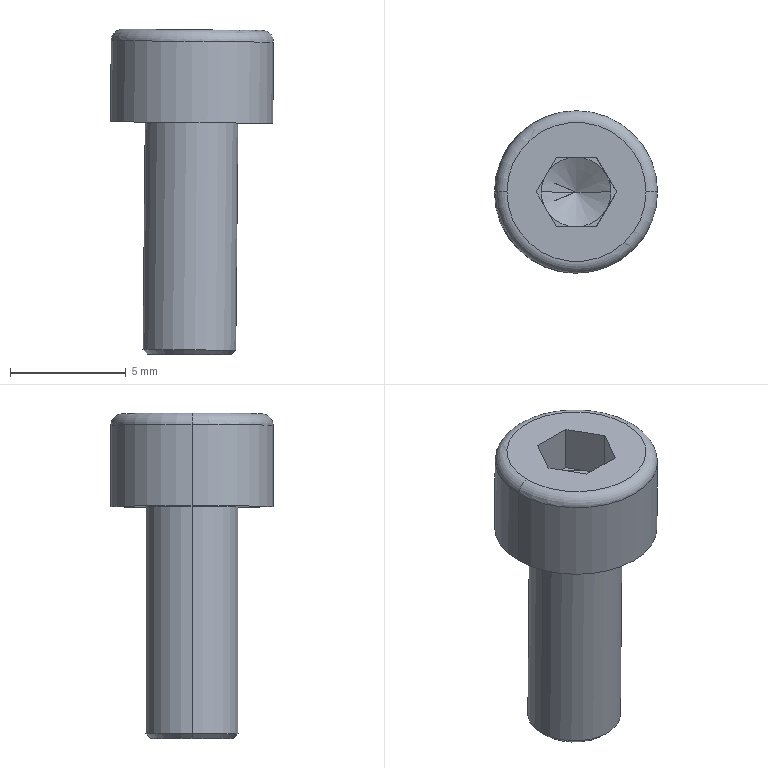Component | SolidWorks | hexagon socket head cap screws gb-14 | 1 solid | 25 faces | box 7.03 x 7 x 14.05 mm | volume 261 mm3 | plane 15 | cone 4 | cylinder 4 | torus 2 | commonest cylinder face diameters 4 x2 7 x2
STEP:
#1=CARTESIAN_POINT('',(-0.8105,1.397,-0.0293));
#2=VERTEX_POINT('',#1);
#3=CARTESIAN_POINT('',(-0.6688,1.397,-0.03069));
#4=VERTEX_POINT('',#3);
#5=CARTESIAN_POINT('',(-0.7397,1.397,-0.03));
#6=DIRECTION('',(-0.009793,0.,-1.));
#7=DIRECTION('',(-1.,0.,0.009793));
#8=AXIS2_PLACEMENT_3D('',#5,#6,#7);
#9=CIRCLE('',#8,0.07087);
#10=EDGE_CURVE('',#2,#4,#9,.T.);
#11=ORIENTED_EDGE('',*,*,#10,.F.);
#12=CARTESIAN_POINT('',(-0.8183,1.397,-0.02135));
#13=VERTEX_POINT('',#12);
#14=CARTESIAN_POINT('',(-0.8105,1.397,-0.0293));
#15=DIRECTION('',(-0.7001,-0.,0.714));
#16=VECTOR('',#15,39.37);
#17=LINE('',#14,#16);
#18=EDGE_CURVE('',#2,#13,#17,.T.);
#19=ORIENTED_EDGE('',*,*,#18,.T.);
#20=CARTESIAN_POINT('',(-0.6609,1.397,-0.02289));
#21=VERTEX_POINT('',#20);
#22=CARTESIAN_POINT('',(-0.7396,1.397,-0.02212));
#23=DIRECTION('',(0.009793,-0.,1.));
#24=DIRECTION('',(-1.,0.,0.009793));
#25=AXIS2_PLACEMENT_3D('',#22,#23,#24);
#26=CIRCLE('',#25,0.07874);
#27=EDGE_CURVE('',#21,#13,#26,.T.);
#28=ORIENTED_EDGE('',*,*,#27,.F.);
#29=CARTESIAN_POINT('',(-0.6688,1.397,-0.03069));
#30=DIRECTION('',(0.714,-0.,0.7001));
#31=VECTOR('',#30,39.37);
#32=LINE('',#29,#31);
#33=EDGE_CURVE('',#4,#21,#32,.T.);
#34=ORIENTED_EDGE('',*,*,#33,.F.);
#35=EDGE_LOOP('',(#11,#19,#28,#34));
#36=FACE_OUTER_BOUND('',#35,.T.);
#37=CARTESIAN_POINT('',(-0.7397,1.397,-0.03));
#38=DIRECTION('',(0.009793,-0.,1.));
#39=DIRECTION('',(1.,0.,-0.009793));
#40=AXIS2_PLACEMENT_3D('',#37,#38,#39);
#41=CONICAL_SURFACE('',#40,0.07087,0.7854);
#42=ADVANCED_FACE('',(#36),#41,.T.);
#43=CARTESIAN_POINT('',(-0.6162,1.397,0.52));
#44=VERTEX_POINT('',#43);
#45=CARTESIAN_POINT('',(-0.8524,1.397,0.5223));
#46=VERTEX_POINT('',#45);
#47=CARTESIAN_POINT('',(-0.7343,1.397,0.5212));
#48=DIRECTION('',(0.009793,-0.,1.));
#49=DIRECTION('',(-1.,0.,0.009793));
#50=AXIS2_PLACEMENT_3D('',#47,#48,#49);
#51=CIRCLE('',#50,0.1181);
#52=EDGE_CURVE('',#44,#46,#51,.T.);
#53=ORIENTED_EDGE('',*,*,#52,.F.);
#54=CARTESIAN_POINT('',(-0.5967,1.397,0.5001));
#55=VERTEX_POINT('',#54);
#56=CARTESIAN_POINT('',(-0.6164,1.397,0.5003));
#57=DIRECTION('',(-0.,1.,0.));
#58=DIRECTION('',(0.,0.,1.));
#59=AXIS2_PLACEMENT_3D('',#56,#57,#58);
#60=CIRCLE('',#59,0.01969);
#61=EDGE_CURVE('',#44,#55,#60,.T.);
#62=ORIENTED_EDGE('',*,*,#61,.T.);
#63=CARTESIAN_POINT('',(-0.8723,1.397,0.5028));
#64=VERTEX_POINT('',#63);
#65=CARTESIAN_POINT('',(-0.7345,1.397,0.5015));
#66=DIRECTION('',(-0.009793,0.,-1.));
#67=DIRECTION('',(-1.,0.,0.009793));
#68=AXIS2_PLACEMENT_3D('',#65,#66,#67);
#69=CIRCLE('',#68,0.1378);
#70=EDGE_CURVE('',#64,#55,#69,.T.);
#71=ORIENTED_EDGE('',*,*,#70,.F.);
#72=CARTESIAN_POINT('',(-0.8526,1.397,0.5026));
#73=DIRECTION('',(0.,-1.,-0.));
#74=DIRECTION('',(0.,0.,-1.));
#75=AXIS2_PLACEMENT_3D('',#72,#73,#74);
#76=CIRCLE('',#75,0.01969);
#77=EDGE_CURVE('',#46,#64,#76,.T.);
#78=ORIENTED_EDGE('',*,*,#77,.F.);
#79=EDGE_LOOP('',(#53,#62,#71,#78));
#80=FACE_OUTER_BOUND('',#79,.T.);
#81=CARTESIAN_POINT('',(-0.7345,1.397,0.5015));
#82=DIRECTION('',(-0.009793,0.,-1.));
#83=DIRECTION('',(-1.,0.,0.009793));
#84=AXIS2_PLACEMENT_3D('',#81,#82,#83);
#85=TOROIDAL_SURFACE('',#84,0.1181,0.01969);
#86=ADVANCED_FACE('',(#80),#85,.T.);
#87=CARTESIAN_POINT('',(-0.7354,1.397,0.4083));
#88=VERTEX_POINT('',#87);
#89=CARTESIAN_POINT('',(-0.676,1.397,0.4418));
#90=VERTEX_POINT('',#89);
#91=CARTESIAN_POINT('',(-0.676,1.397,0.4418));
#92=DIRECTION('',(0.8709,-0.,0.4915));
#93=VECTOR('',#92,39.37);
#94=LINE('',#91,#93);
#95=EDGE_CURVE('',#88,#90,#94,.T.);
#96=ORIENTED_EDGE('',*,*,#95,.F.);
#97=CARTESIAN_POINT('',(-0.7941,1.397,0.443));
#98=VERTEX_POINT('',#97);
#99=CARTESIAN_POINT('',(-0.7941,1.397,0.443));
#100=DIRECTION('',(-0.8611,-0.,0.5085));
#101=VECTOR('',#100,39.37);
#102=LINE('',#99,#101);
#103=EDGE_CURVE('',#88,#98,#102,.T.);
#104=ORIENTED_EDGE('',*,*,#103,.T.);
#105=CARTESIAN_POINT('',(-0.7862,1.368,0.4429));
#106=VERTEX_POINT('',#105);
#107=CARTESIAN_POINT('',(-0.7351,1.397,0.4424));
#108=DIRECTION('',(-0.009793,0.,-1.));
#109=DIRECTION('',(1.,0.,-0.009793));
#110=AXIS2_PLACEMENT_3D('',#107,#108,#109);
#111=CIRCLE('',#110,0.05906);
#112=EDGE_CURVE('',#106,#98,#111,.T.);
#113=ORIENTED_EDGE('',*,*,#112,.F.);
#114=CARTESIAN_POINT('',(-0.7351,1.338,0.4424));
#115=VERTEX_POINT('',#114);
#116=CARTESIAN_POINT('',(-0.7351,1.397,0.4424));
#117=DIRECTION('',(-0.009793,0.,-1.));
#118=DIRECTION('',(1.,0.,-0.009793));
#119=AXIS2_PLACEMENT_3D('',#116,#117,#118);
#120=CIRCLE('',#119,0.05906);
#121=EDGE_CURVE('',#115,#106,#120,.T.);
#122=ORIENTED_EDGE('',*,*,#121,.F.);
#123=CARTESIAN_POINT('',(-0.6839,1.368,0.4419));
#124=VERTEX_POINT('',#123);
#125=CARTESIAN_POINT('',(-0.7351,1.397,0.4424));
#126=DIRECTION('',(-0.009793,0.,-1.));
#127=DIRECTION('',(1.,0.,-0.009793));
#128=AXIS2_PLACEMENT_3D('',#125,#126,#127);
#129=CIRCLE('',#128,0.05906);
#130=EDGE_CURVE('',#124,#115,#129,.T.);
#131=ORIENTED_EDGE('',*,*,#130,.F.);
#132=CARTESIAN_POINT('',(-0.7351,1.397,0.4424));
#133=DIRECTION('',(-0.009793,0.,-1.));
#134=DIRECTION('',(1.,0.,-0.009793));
#135=AXIS2_PLACEMENT_3D('',#132,#133,#134);
#136=CIRCLE('',#135,0.05906);
#137=EDGE_CURVE('',#90,#124,#136,.T.);
#138=ORIENTED_EDGE('',*,*,#137,.F.);
#139=EDGE_LOOP('',(#96,#104,#113,#122,#131,#138));
#140=FACE_OUTER_BOUND('',#139,.T.);
#141=CARTESIAN_POINT('',(-0.7351,1.397,0.4424));
#142=DIRECTION('',(0.009793,-0.,1.));
#143=DIRECTION('',(1.,0.,-0.009793));
#144=AXIS2_PLACEMENT_3D('',#141,#142,#143);
#145=CONICAL_SURFACE('',#144,0.05906,1.047);
#146=ADVANCED_FACE('',(#140),#145,.F.);
#147=ORIENTED_EDGE('',*,*,#27,.T.);
#148=CARTESIAN_POINT('',(-0.8146,1.397,0.3645));
#149=VERTEX_POINT('',#148);
#150=CARTESIAN_POINT('',(-0.8184,1.397,-0.02923));
#151=DIRECTION('',(0.009793,-0.,1.));
#152=VECTOR('',#151,39.37);
#153=LINE('',#150,#152);
#154=EDGE_CURVE('',#13,#149,#153,.T.);
#155=ORIENTED_EDGE('',*,*,#154,.T.);
#156=CARTESIAN_POINT('',(-0.6571,1.397,0.3629));
#157=VERTEX_POINT('',#156);
#158=CARTESIAN_POINT('',(-0.7358,1.397,0.3637));
#159=DIRECTION('',(-0.009793,0.,-1.));
#160=DIRECTION('',(-1.,0.,0.009793));
#161=AXIS2_PLACEMENT_3D('',#158,#159,#160);
#162=CIRCLE('',#161,0.07874);
#163=EDGE_CURVE('',#149,#157,#162,.T.);
#164=ORIENTED_EDGE('',*,*,#163,.T.);
#165=CARTESIAN_POINT('',(-0.661,1.397,-0.03077));
#166=DIRECTION('',(0.009793,-0.,1.));
#167=VECTOR('',#166,39.37);
#168=LINE('',#165,#167);
#169=EDGE_CURVE('',#21,#157,#168,.T.);
#170=ORIENTED_EDGE('',*,*,#169,.F.);
#171=EDGE_LOOP('',(#147,#155,#164,#170));
#172=FACE_OUTER_BOUND('',#171,.T.);
#173=CARTESIAN_POINT('',(-0.7397,1.397,-0.03));
#174=DIRECTION('',(0.009793,-0.,1.));
#175=DIRECTION('',(1.,0.,-0.009793));
#176=AXIS2_PLACEMENT_3D('',#173,#174,#175);
#177=CYLINDRICAL_SURFACE('',#176,0.07874);
#178=ADVANCED_FACE('',(#172),#177,.T.);
#179=CARTESIAN_POINT('',(-0.8736,1.397,0.365));
#180=VERTEX_POINT('',#179);
#181=CARTESIAN_POINT('',(-0.598,1.397,0.3623));
#182=VERTEX_POINT('',#181);
#183=CARTESIAN_POINT('',(-0.7358,1.397,0.3637));
#184=DIRECTION('',(-0.009793,0.,-1.));
#185=DIRECTION('',(-1.,0.,0.009793));
#186=AXIS2_PLACEMENT_3D('',#183,#184,#185);
#187=CIRCLE('',#186,0.1378);
#188=EDGE_CURVE('',#180,#182,#187,.T.);
#189=ORIENTED_EDGE('',*,*,#188,.F.);
#190=CARTESIAN_POINT('',(-0.8736,1.397,0.365));
#191=DIRECTION('',(0.009793,-0.,1.));
#192=VECTOR('',#191,39.37);
#193=LINE('',#190,#192);
#194=EDGE_CURVE('',#180,#64,#193,.T.);
#195=ORIENTED_EDGE('',*,*,#194,.T.);
#196=ORIENTED_EDGE('',*,*,#70,.T.);
#197=CARTESIAN_POINT('',(-0.598,1.397,0.3623));
#198=DIRECTION('',(0.009793,-0.,1.));
#199=VECTOR('',#198,39.37);
#200=LINE('',#197,#199);
#201=EDGE_CURVE('',#182,#55,#200,.T.);
#202=ORIENTED_EDGE('',*,*,#201,.F.);
#203=EDGE_LOOP('',(#189,#195,#196,#202));
#204=FACE_OUTER_BOUND('',#203,.T.);
#205=CARTESIAN_POINT('',(-0.7358,1.397,0.3637));
#206=DIRECTION('',(0.009793,-0.,1.));
#207=DIRECTION('',(1.,0.,-0.009793));
#208=AXIS2_PLACEMENT_3D('',#205,#206,#207);
#209=CYLINDRICAL_SURFACE('',#208,0.1378);
#210=ADVANCED_FACE('',(#204),#209,.T.);
#211=CARTESIAN_POINT('',(-0.701,1.338,0.4421));
#212=VERTEX_POINT('',#211);
#213=CARTESIAN_POINT('',(-0.6669,1.397,0.4418));
#214=DIRECTION('',(-0.5,-0.866,0.004897));
#215=VECTOR('',#214,39.37);
#216=LINE('',#213,#215);
#217=EDGE_CURVE('',#124,#212,#216,.T.);
#218=ORIENTED_EDGE('',*,*,#217,.F.);
#219=ORIENTED_EDGE('',*,*,#130,.T.);
#220=CARTESIAN_POINT('',(-0.701,1.338,0.4421));
#221=DIRECTION('',(-1.,-0.,0.009793));
#222=VECTOR('',#221,39.37);
#223=LINE('',#220,#222);
#224=EDGE_CURVE('',#212,#115,#223,.T.);
#225=ORIENTED_EDGE('',*,*,#224,.F.);
#226=EDGE_LOOP('',(#218,#219,#225));
#227=FACE_OUTER_BOUND('',#226,.T.);
#228=CARTESIAN_POINT('',(-0.7351,1.279,0.4424));
#229=DIRECTION('',(0.009793,-0.,1.));
#230=DIRECTION('',(1.,0.,-0.009793));
#231=AXIS2_PLACEMENT_3D('',#228,#229,#230);
#232=PLANE('',#231);
#233=ADVANCED_FACE('',(#227),#232,.T.);
#234=CARTESIAN_POINT('',(-0.7692,1.338,0.4428));
#235=VERTEX_POINT('',#234);
#236=CARTESIAN_POINT('',(-0.701,1.338,0.4421));
#237=DIRECTION('',(-1.,-0.,0.009793));
#238=VECTOR('',#237,39.37);
#239=LINE('',#236,#238);
#240=EDGE_CURVE('',#115,#235,#239,.T.);
#241=ORIENTED_EDGE('',*,*,#240,.F.);
#242=ORIENTED_EDGE('',*,*,#121,.T.);
#243=CARTESIAN_POINT('',(-0.7692,1.338,0.4428));
#244=DIRECTION('',(-0.5,0.866,0.004897));
#245=VECTOR('',#244,39.37);
#246=LINE('',#243,#245);
#247=EDGE_CURVE('',#235,#106,#246,.T.);
#248=ORIENTED_EDGE('',*,*,#247,.F.);
#249=EDGE_LOOP('',(#241,#242,#248));
#250=FACE_OUTER_BOUND('',#249,.T.);
#251=CARTESIAN_POINT('',(-0.7351,1.279,0.4424));
#252=DIRECTION('',(0.009793,-0.,1.));
#253=DIRECTION('',(1.,0.,-0.009793));
#254=AXIS2_PLACEMENT_3D('',#251,#252,#253);
#255=PLANE('',#254);
#256=ADVANCED_FACE('',(#250),#255,.T.);
#257=CARTESIAN_POINT('',(-0.8032,1.397,0.4431));
#258=VERTEX_POINT('',#257);
#259=CARTESIAN_POINT('',(-0.7692,1.338,0.4428));
#260=DIRECTION('',(-0.5,0.866,0.004897));
#261=VECTOR('',#260,39.37);
#262=LINE('',#259,#261);
#263=EDGE_CURVE('',#106,#258,#262,.T.);
#264=ORIENTED_EDGE('',*,*,#263,.F.);
#265=ORIENTED_EDGE('',*,*,#112,.T.);
#266=CARTESIAN_POINT('',(-0.7862,1.427,0.4429));
#267=VERTEX_POINT('',#266);
#268=CARTESIAN_POINT('',(-0.7351,1.397,0.4424));
#269=DIRECTION('',(-0.009793,0.,-1.));
#270=DIRECTION('',(1.,0.,-0.009793));
#271=AXIS2_PLACEMENT_3D('',#268,#269,#270);
#272=CIRCLE('',#271,0.05906);
#273=EDGE_CURVE('',#98,#267,#272,.T.);
#274=ORIENTED_EDGE('',*,*,#273,.T.);
#275=CARTESIAN_POINT('',(-0.8032,1.397,0.4431));
#276=DIRECTION('',(0.5,0.866,-0.004897));
#277=VECTOR('',#276,39.37);
#278=LINE('',#275,#277);
#279=EDGE_CURVE('',#258,#267,#278,.T.);
#280=ORIENTED_EDGE('',*,*,#279,.F.);
#281=EDGE_LOOP('',(#264,#265,#274,#280));
#282=FACE_OUTER_BOUND('',#281,.T.);
#283=CARTESIAN_POINT('',(-0.7351,1.279,0.4424));
#284=DIRECTION('',(0.009793,-0.,1.));
#285=DIRECTION('',(1.,0.,-0.009793));
#286=AXIS2_PLACEMENT_3D('',#283,#284,#285);
#287=PLANE('',#286);
#288=ADVANCED_FACE('',(#282),#287,.T.);
#289=CARTESIAN_POINT('',(-0.7692,1.456,0.4428));
#290=VERTEX_POINT('',#289);
#291=CARTESIAN_POINT('',(-0.8032,1.397,0.4431));
#292=DIRECTION('',(0.5,0.866,-0.004897));
#293=VECTOR('',#292,39.37);
#294=LINE('',#291,#293);
#295=EDGE_CURVE('',#267,#290,#294,.T.);
#296=ORIENTED_EDGE('',*,*,#295,.F.);
#297=CARTESIAN_POINT('',(-0.7351,1.456,0.4424));
#298=VERTEX_POINT('',#297);
#299=CARTESIAN_POINT('',(-0.7351,1.397,0.4424));
#300=DIRECTION('',(-0.009793,0.,-1.));
#301=DIRECTION('',(-1.,0.,0.009793));
#302=AXIS2_PLACEMENT_3D('',#299,#300,#301);
#303=CIRCLE('',#302,0.05906);
#304=EDGE_CURVE('',#267,#298,#303,.T.);
#305=ORIENTED_EDGE('',*,*,#304,.T.);
#306=CARTESIAN_POINT('',(-0.7692,1.456,0.4428));
#307=DIRECTION('',(1.,0.,-0.009793));
#308=VECTOR('',#307,39.37);
#309=LINE('',#306,#308);
#310=EDGE_CURVE('',#290,#298,#309,.T.);
#311=ORIENTED_EDGE('',*,*,#310,.F.);
#312=EDGE_LOOP('',(#296,#305,#311));
#313=FACE_OUTER_BOUND('',#312,.T.);
#314=CARTESIAN_POINT('',(-0.7351,1.279,0.4424));
#315=DIRECTION('',(0.009793,-0.,1.));
#316=DIRECTION('',(1.,0.,-0.009793));
#317=AXIS2_PLACEMENT_3D('',#314,#315,#316);
#318=PLANE('',#317);
#319=ADVANCED_FACE('',(#313),#318,.T.);
#320=CARTESIAN_POINT('',(-0.701,1.456,0.4421));
#321=VERTEX_POINT('',#320);
#322=CARTESIAN_POINT('',(-0.7692,1.456,0.4428));
#323=DIRECTION('',(1.,0.,-0.009793));
#324=VECTOR('',#323,39.37);
#325=LINE('',#322,#324);
#326=EDGE_CURVE('',#298,#321,#325,.T.);
#327=ORIENTED_EDGE('',*,*,#326,.F.);
#328=CARTESIAN_POINT('',(-0.6839,1.427,0.4419));
#329=VERTEX_POINT('',#328);
#330=CARTESIAN_POINT('',(-0.7351,1.397,0.4424));
#331=DIRECTION('',(-0.009793,0.,-1.));
#332=DIRECTION('',(1.,0.,-0.009793));
#333=AXIS2_PLACEMENT_3D('',#330,#331,#332);
#334=CIRCLE('',#333,0.05906);
#335=EDGE_CURVE('',#298,#329,#334,.T.);
#336=ORIENTED_EDGE('',*,*,#335,.T.);
#337=CARTESIAN_POINT('',(-0.701,1.456,0.4421));
#338=DIRECTION('',(0.5,-0.866,-0.004897));
#339=VECTOR('',#338,39.37);
#340=LINE('',#337,#339);
#341=EDGE_CURVE('',#321,#329,#340,.T.);
#342=ORIENTED_EDGE('',*,*,#341,.F.);
#343=EDGE_LOOP('',(#327,#336,#342));
#344=FACE_OUTER_BOUND('',#343,.T.);
#345=CARTESIAN_POINT('',(-0.7351,1.279,0.4424));
#346=DIRECTION('',(0.009793,-0.,1.));
#347=DIRECTION('',(1.,0.,-0.009793));
#348=AXIS2_PLACEMENT_3D('',#345,#346,#347);
#349=PLANE('',#348);
#350=ADVANCED_FACE('',(#344),#349,.T.);
#351=CARTESIAN_POINT('',(-0.6669,1.397,0.4418));
#352=VERTEX_POINT('',#351);
#353=CARTESIAN_POINT('',(-0.701,1.456,0.4421));
#354=DIRECTION('',(0.5,-0.866,-0.004897));
#355=VECTOR('',#354,39.37);
#356=LINE('',#353,#355);
#357=EDGE_CURVE('',#329,#352,#356,.T.);
#358=ORIENTED_EDGE('',*,*,#357,.F.);
#359=CARTESIAN_POINT('',(-0.7351,1.397,0.4424));
#360=DIRECTION('',(-0.009793,0.,-1.));
#361=DIRECTION('',(1.,0.,-0.009793));
#362=AXIS2_PLACEMENT_3D('',#359,#360,#361);
#363=CIRCLE('',#362,0.05906);
#364=EDGE_CURVE('',#329,#90,#363,.T.);
#365=ORIENTED_EDGE('',*,*,#364,.T.);
#366=ORIENTED_EDGE('',*,*,#137,.T.);
#367=CARTESIAN_POINT('',(-0.6669,1.397,0.4418));
#368=DIRECTION('',(-0.5,-0.866,0.004897));
#369=VECTOR('',#368,39.37);
#370=LINE('',#367,#369);
#371=EDGE_CURVE('',#352,#124,#370,.T.);
#372=ORIENTED_EDGE('',*,*,#371,.F.);
#373=EDGE_LOOP('',(#358,#365,#366,#372));
#374=FACE_OUTER_BOUND('',#373,.T.);
#375=CARTESIAN_POINT('',(-0.7351,1.279,0.4424));
#376=DIRECTION('',(0.009793,-0.,1.));
#377=DIRECTION('',(1.,0.,-0.009793));
#378=AXIS2_PLACEMENT_3D('',#375,#376,#377);
#379=PLANE('',#378);
#380=ADVANCED_FACE('',(#374),#379,.T.);
#381=CARTESIAN_POINT('',(-0.7343,1.397,0.5212));
#382=DIRECTION('',(0.009793,-0.,1.));
#383=DIRECTION('',(-1.,0.,0.009793));
#384=AXIS2_PLACEMENT_3D('',#381,#382,#383);
#385=CIRCLE('',#384,0.1181);
#386=EDGE_CURVE('',#46,#44,#385,.T.);
#387=ORIENTED_EDGE('',*,*,#386,.T.);
#388=ORIENTED_EDGE('',*,*,#52,.T.);
#389=EDGE_LOOP('',(#387,#388));
#390=FACE_OUTER_BOUND('',#389,.T.);
#391=CARTESIAN_POINT('',(-0.7684,1.338,0.5215));
#392=VERTEX_POINT('',#391);
#393=CARTESIAN_POINT('',(-0.8025,1.397,0.5218));
#394=VERTEX_POINT('',#393);
#395=CARTESIAN_POINT('',(-0.7684,1.338,0.5215));
#396=DIRECTION('',(-0.5,0.866,0.004897));
#397=VECTOR('',#396,39.37);
#398=LINE('',#395,#397);
#399=EDGE_CURVE('',#392,#394,#398,.T.);
#400=ORIENTED_EDGE('',*,*,#399,.T.);
#401=CARTESIAN_POINT('',(-0.7684,1.456,0.5215));
#402=VERTEX_POINT('',#401);
#403=CARTESIAN_POINT('',(-0.8025,1.397,0.5218));
#404=DIRECTION('',(0.5,0.866,-0.004897));
#405=VECTOR('',#404,39.37);
#406=LINE('',#403,#405);
#407=EDGE_CURVE('',#394,#402,#406,.T.);
#408=ORIENTED_EDGE('',*,*,#407,.T.);
#409=CARTESIAN_POINT('',(-0.7002,1.456,0.5208));
#410=VERTEX_POINT('',#409);
#411=CARTESIAN_POINT('',(-0.7684,1.456,0.5215));
#412=DIRECTION('',(1.,0.,-0.009793));
#413=VECTOR('',#412,39.37);
#414=LINE('',#411,#413);
#415=EDGE_CURVE('',#402,#410,#414,.T.);
#416=ORIENTED_EDGE('',*,*,#415,.T.);
#417=CARTESIAN_POINT('',(-0.6661,1.397,0.5205));
#418=VERTEX_POINT('',#417);
#419=CARTESIAN_POINT('',(-0.7002,1.456,0.5208));
#420=DIRECTION('',(0.5,-0.866,-0.004897));
#421=VECTOR('',#420,39.37);
#422=LINE('',#419,#421);
#423=EDGE_CURVE('',#410,#418,#422,.T.);
#424=ORIENTED_EDGE('',*,*,#423,.T.);
#425=CARTESIAN_POINT('',(-0.7002,1.338,0.5208));
#426=VERTEX_POINT('',#425);
#427=CARTESIAN_POINT('',(-0.6661,1.397,0.5205));
#428=DIRECTION('',(-0.5,-0.866,0.004897));
#429=VECTOR('',#428,39.37);
#430=LINE('',#427,#429);
#431=EDGE_CURVE('',#418,#426,#430,.T.);
#432=ORIENTED_EDGE('',*,*,#431,.T.);
#433=CARTESIAN_POINT('',(-0.7002,1.338,0.5208));
#434=DIRECTION('',(-1.,-0.,0.009793));
#435=VECTOR('',#434,39.37);
#436=LINE('',#433,#435);
#437=EDGE_CURVE('',#426,#392,#436,.T.);
#438=ORIENTED_EDGE('',*,*,#437,.T.);
#439=EDGE_LOOP('',(#400,#408,#416,#424,#432,#438));
#440=FACE_BOUND('',#439,.T.);
#441=CARTESIAN_POINT('',(-0.7343,1.397,0.5212));
#442=DIRECTION('',(-0.009793,0.,-1.));
#443=DIRECTION('',(-1.,-0.,0.009793));
#444=AXIS2_PLACEMENT_3D('',#441,#442,#443);
#445=PLANE('',#444);
#446=ADVANCED_FACE('',(#390,#440),#445,.F.);
#447=CARTESIAN_POINT('',(-0.7358,1.397,0.3637));
#448=DIRECTION('',(-0.009793,0.,-1.));
#449=DIRECTION('',(-1.,0.,0.009793));
#450=AXIS2_PLACEMENT_3D('',#447,#448,#449);
#451=CIRCLE('',#450,0.1378);
#452=EDGE_CURVE('',#182,#180,#451,.T.);
#453=ORIENTED_EDGE('',*,*,#452,.T.);
#454=ORIENTED_EDGE('',*,*,#188,.T.);
#455=EDGE_LOOP('',(#453,#454));
#456=FACE_OUTER_BOUND('',#455,.T.);
#457=CARTESIAN_POINT('',(-0.7358,1.397,0.3637));
#458=DIRECTION('',(-0.009793,0.,-1.));
#459=DIRECTION('',(-1.,0.,0.009793));
#460=AXIS2_PLACEMENT_3D('',#457,#458,#459);
#461=CIRCLE('',#460,0.07874);
#462=EDGE_CURVE('',#157,#149,#461,.T.);
#463=ORIENTED_EDGE('',*,*,#462,.F.);
#464=ORIENTED_EDGE('',*,*,#163,.F.);
#465=EDGE_LOOP('',(#463,#464));
#466=FACE_BOUND('',#465,.T.);
#467=CARTESIAN_POINT('',(-0.7358,1.397,0.3637));
#468=DIRECTION('',(-0.009793,0.,-1.));
#469=DIRECTION('',(-1.,-0.,0.009793));
#470=AXIS2_PLACEMENT_3D('',#467,#468,#469);
#471=PLANE('',#470);
#472=ADVANCED_FACE('',(#456,#466),#471,.T.);
#473=ORIENTED_EDGE('',*,*,#194,.F.);
#474=ORIENTED_EDGE('',*,*,#452,.F.);
#475=ORIENTED_EDGE('',*,*,#201,.T.);
#476=CARTESIAN_POINT('',(-0.7345,1.397,0.5015));
#477=DIRECTION('',(-0.009793,0.,-1.));
#478=DIRECTION('',(-1.,0.,0.009793));
#479=AXIS2_PLACEMENT_3D('',#476,#477,#478);
#480=CIRCLE('',#479,0.1378);
#481=EDGE_CURVE('',#55,#64,#480,.T.);
#482=ORIENTED_EDGE('',*,*,#481,.T.);
#483=EDGE_LOOP('',(#473,#474,#475,#482));
#484=FACE_OUTER_BOUND('',#483,.T.);
#485=CARTESIAN_POINT('',(-0.7358,1.397,0.3637));
#486=DIRECTION('',(0.009793,-0.,1.));
#487=DIRECTION('',(1.,0.,-0.009793));
#488=AXIS2_PLACEMENT_3D('',#485,#486,#487);
#489=CYLINDRICAL_SURFACE('',#488,0.1378);
#490=ADVANCED_FACE('',(#484),#489,.T.);
#491=ORIENTED_EDGE('',*,*,#154,.F.);
#492=CARTESIAN_POINT('',(-0.7396,1.397,-0.02212));
#493=DIRECTION('',(0.009793,-0.,1.));
#494=DIRECTION('',(-1.,0.,0.009793));
#495=AXIS2_PLACEMENT_3D('',#492,#493,#494);
#496=CIRCLE('',#495,0.07874);
#497=EDGE_CURVE('',#13,#21,#496,.T.);
#498=ORIENTED_EDGE('',*,*,#497,.T.);
#499=ORIENTED_EDGE('',*,*,#169,.T.);
#500=ORIENTED_EDGE('',*,*,#462,.T.);
#501=EDGE_LOOP('',(#491,#498,#499,#500));
#502=FACE_OUTER_BOUND('',#501,.T.);
#503=CARTESIAN_POINT('',(-0.7397,1.397,-0.03));
#504=DIRECTION('',(0.009793,-0.,1.));
#505=DIRECTION('',(1.,0.,-0.009793));
#506=AXIS2_PLACEMENT_3D('',#503,#504,#505);
#507=CYLINDRICAL_SURFACE('',#506,0.07874);
#508=ADVANCED_FACE('',(#502),#507,.T.);
#509=CARTESIAN_POINT('',(-0.7397,1.397,-0.03));
#510=DIRECTION('',(-0.009793,0.,-1.));
#511=DIRECTION('',(-1.,0.,0.009793));
#512=AXIS2_PLACEMENT_3D('',#509,#510,#511);
#513=CIRCLE('',#512,0.07087);
#514=EDGE_CURVE('',#4,#2,#513,.T.);
#515=ORIENTED_EDGE('',*,*,#514,.T.);
#516=ORIENTED_EDGE('',*,*,#10,.T.);
#517=EDGE_LOOP('',(#515,#516));
#518=FACE_OUTER_BOUND('',#517,.T.);
#519=CARTESIAN_POINT('',(-0.7397,1.397,-0.03));
#520=DIRECTION('',(-0.009793,0.,-1.));
#521=DIRECTION('',(-1.,-0.,0.009793));
#522=AXIS2_PLACEMENT_3D('',#519,#520,#521);
#523=PLANE('',#522);
#524=ADVANCED_FACE('',(#518),#523,.T.);
#525=ORIENTED_EDGE('',*,*,#399,.F.);
#526=CARTESIAN_POINT('',(-0.7692,1.338,0.4428));
#527=DIRECTION('',(0.009793,-0.,1.));
#528=VECTOR('',#527,39.37);
#529=LINE('',#526,#528);
#530=EDGE_CURVE('',#235,#392,#529,.T.);
#531=ORIENTED_EDGE('',*,*,#530,.F.);
#532=ORIENTED_EDGE('',*,*,#247,.T.);
#533=ORIENTED_EDGE('',*,*,#263,.T.);
#534=CARTESIAN_POINT('',(-0.8032,1.397,0.4431));
#535=DIRECTION('',(0.009793,-0.,1.));
#536=VECTOR('',#535,39.37);
#537=LINE('',#534,#536);
#538=EDGE_CURVE('',#258,#394,#537,.T.);
#539=ORIENTED_EDGE('',*,*,#538,.T.);
#540=EDGE_LOOP('',(#525,#531,#532,#533,#539));
#541=FACE_OUTER_BOUND('',#540,.T.);
#542=CARTESIAN_POINT('',(-0.7692,1.338,0.4428));
#543=DIRECTION('',(0.866,0.5,-0.008481));
#544=DIRECTION('',(0.5,-0.866,-0.004897));
#545=AXIS2_PLACEMENT_3D('',#542,#543,#544);
#546=PLANE('',#545);
#547=ADVANCED_FACE('',(#541),#546,.T.);
#548=ORIENTED_EDGE('',*,*,#407,.F.);
#549=ORIENTED_EDGE('',*,*,#538,.F.);
#550=ORIENTED_EDGE('',*,*,#279,.T.);
#551=ORIENTED_EDGE('',*,*,#295,.T.);
#552=CARTESIAN_POINT('',(-0.7692,1.456,0.4428));
#553=DIRECTION('',(0.009793,-0.,1.));
#554=VECTOR('',#553,39.37);
#555=LINE('',#552,#554);
#556=EDGE_CURVE('',#290,#402,#555,.T.);
#557=ORIENTED_EDGE('',*,*,#556,.T.);
#558=EDGE_LOOP('',(#548,#549,#550,#551,#557));
#559=FACE_OUTER_BOUND('',#558,.T.);
#560=CARTESIAN_POINT('',(-0.8032,1.397,0.4431));
#561=DIRECTION('',(0.866,-0.5,-0.008481));
#562=DIRECTION('',(-0.5,-0.866,0.004897));
#563=AXIS2_PLACEMENT_3D('',#560,#561,#562);
#564=PLANE('',#563);
#565=ADVANCED_FACE('',(#559),#564,.T.);
#566=ORIENTED_EDGE('',*,*,#415,.F.);
#567=ORIENTED_EDGE('',*,*,#556,.F.);
#568=ORIENTED_EDGE('',*,*,#310,.T.);
#569=ORIENTED_EDGE('',*,*,#326,.T.);
#570=CARTESIAN_POINT('',(-0.701,1.456,0.4421));
#571=DIRECTION('',(0.009793,-0.,1.));
#572=VECTOR('',#571,39.37);
#573=LINE('',#570,#572);
#574=EDGE_CURVE('',#321,#410,#573,.T.);
#575=ORIENTED_EDGE('',*,*,#574,.T.);
#576=EDGE_LOOP('',(#566,#567,#568,#569,#575));
#577=FACE_OUTER_BOUND('',#576,.T.);
#578=CARTESIAN_POINT('',(-0.7692,1.456,0.4428));
#579=DIRECTION('',(0.,-1.,-0.));
#580=DIRECTION('',(-1.,-0.,0.009793));
#581=AXIS2_PLACEMENT_3D('',#578,#579,#580);
#582=PLANE('',#581);
#583=ADVANCED_FACE('',(#577),#582,.T.);
#584=ORIENTED_EDGE('',*,*,#423,.F.);
#585=ORIENTED_EDGE('',*,*,#574,.F.);
#586=ORIENTED_EDGE('',*,*,#341,.T.);
#587=ORIENTED_EDGE('',*,*,#357,.T.);
#588=CARTESIAN_POINT('',(-0.6669,1.397,0.4418));
#589=DIRECTION('',(0.009793,-0.,1.));
#590=VECTOR('',#589,39.37);
#591=LINE('',#588,#590);
#592=EDGE_CURVE('',#352,#418,#591,.T.);
#593=ORIENTED_EDGE('',*,*,#592,.T.);
#594=EDGE_LOOP('',(#584,#585,#586,#587,#593));
#595=FACE_OUTER_BOUND('',#594,.T.);
#596=CARTESIAN_POINT('',(-0.701,1.456,0.4421));
#597=DIRECTION('',(-0.866,-0.5,0.008481));
#598=DIRECTION('',(-0.5,0.866,0.004897));
#599=AXIS2_PLACEMENT_3D('',#596,#597,#598);
#600=PLANE('',#599);
#601=ADVANCED_FACE('',(#595),#600,.T.);
#602=ORIENTED_EDGE('',*,*,#431,.F.);
#603=ORIENTED_EDGE('',*,*,#592,.F.);
#604=ORIENTED_EDGE('',*,*,#371,.T.);
#605=ORIENTED_EDGE('',*,*,#217,.T.);
#606=CARTESIAN_POINT('',(-0.701,1.338,0.4421));
#607=DIRECTION('',(0.009793,-0.,1.));
#608=VECTOR('',#607,39.37);
#609=LINE('',#606,#608);
#610=EDGE_CURVE('',#212,#426,#609,.T.);
#611=ORIENTED_EDGE('',*,*,#610,.T.);
#612=EDGE_LOOP('',(#602,#603,#604,#605,#611));
#613=FACE_OUTER_BOUND('',#612,.T.);
#614=CARTESIAN_POINT('',(-0.6669,1.397,0.4418));
#615=DIRECTION('',(-0.866,0.5,0.008481));
#616=DIRECTION('',(0.5,0.866,-0.004897));
#617=AXIS2_PLACEMENT_3D('',#614,#615,#616);
#618=PLANE('',#617);
#619=ADVANCED_FACE('',(#613),#618,.T.);
#620=ORIENTED_EDGE('',*,*,#437,.F.);
#621=ORIENTED_EDGE('',*,*,#610,.F.);
#622=ORIENTED_EDGE('',*,*,#224,.T.);
#623=ORIENTED_EDGE('',*,*,#240,.T.);
#624=ORIENTED_EDGE('',*,*,#530,.T.);
#625=EDGE_LOOP('',(#620,#621,#622,#623,#624));
#626=FACE_OUTER_BOUND('',#625,.T.);
#627=CARTESIAN_POINT('',(-0.701,1.338,0.4421));
#628=DIRECTION('',(-0.,1.,0.));
#629=DIRECTION('',(1.,0.,-0.009793));
#630=AXIS2_PLACEMENT_3D('',#627,#628,#629);
#631=PLANE('',#630);
#632=ADVANCED_FACE('',(#626),#631,.T.);
#633=ORIENTED_EDGE('',*,*,#103,.F.);
#634=ORIENTED_EDGE('',*,*,#95,.T.);
#635=ORIENTED_EDGE('',*,*,#364,.F.);
#636=ORIENTED_EDGE('',*,*,#335,.F.);
#637=ORIENTED_EDGE('',*,*,#304,.F.);
#638=ORIENTED_EDGE('',*,*,#273,.F.);
#639=EDGE_LOOP('',(#633,#634,#635,#636,#637,#638));
#640=FACE_OUTER_BOUND('',#639,.T.);
#641=CARTESIAN_POINT('',(-0.7351,1.397,0.4424));
#642=DIRECTION('',(0.009793,-0.,1.));
#643=DIRECTION('',(1.,0.,-0.009793));
#644=AXIS2_PLACEMENT_3D('',#641,#642,#643);
#645=CONICAL_SURFACE('',#644,0.05906,1.047);
#646=ADVANCED_FACE('',(#640),#645,.F.);
#647=ORIENTED_EDGE('',*,*,#61,.F.);
#648=ORIENTED_EDGE('',*,*,#386,.F.);
#649=ORIENTED_EDGE('',*,*,#77,.T.);
#650=ORIENTED_EDGE('',*,*,#481,.F.);
#651=EDGE_LOOP('',(#647,#648,#649,#650));
#652=FACE_OUTER_BOUND('',#651,.T.);
#653=CARTESIAN_POINT('',(-0.7345,1.397,0.5015));
#654=DIRECTION('',(-0.009793,0.,-1.));
#655=DIRECTION('',(-1.,0.,0.009793));
#656=AXIS2_PLACEMENT_3D('',#653,#654,#655);
#657=TOROIDAL_SURFACE('',#656,0.1181,0.01969);
#658=ADVANCED_FACE('',(#652),#657,.T.);
#659=ORIENTED_EDGE('',*,*,#18,.F.);
#660=ORIENTED_EDGE('',*,*,#514,.F.);
#661=ORIENTED_EDGE('',*,*,#33,.T.);
#662=ORIENTED_EDGE('',*,*,#497,.F.);
#663=EDGE_LOOP('',(#659,#660,#661,#662));
#664=FACE_OUTER_BOUND('',#663,.T.);
#665=CARTESIAN_POINT('',(-0.7397,1.397,-0.03));
#666=DIRECTION('',(0.009793,-0.,1.));
#667=DIRECTION('',(1.,0.,-0.009793));
#668=AXIS2_PLACEMENT_3D('',#665,#666,#667);
#669=CONICAL_SURFACE('',#668,0.07087,0.7854);
#670=ADVANCED_FACE('',(#664),#669,.T.);
#671=CLOSED_SHELL('',(#42,#86,#146,#178,#210,#233,#256,#288,#319,#350,#380,#446,#472,#490,#508,#524,#547,#565,#583,#601,#619,#632,#646,#658,#670));
#672=MANIFOLD_SOLID_BREP('',#671);
#673=CARTESIAN_POINT('',(0.,0.,0.));
#674=DIRECTION('',(0.,0.,1.));
#675=DIRECTION('',(1.,0.,0.));
#676=AXIS2_PLACEMENT_3D('',#673,#674,#675);
#677=(LENGTH_UNIT()NAMED_UNIT(*)SI_UNIT($,.METRE.));
#678=LENGTH_MEASURE_WITH_UNIT(LENGTH_MEASURE(0.0254),#677);
#679=DIMENSIONAL_EXPONENTS(1.,0.,0.,0.,0.,0.,0.);
#680=(CONVERSION_BASED_UNIT('',#678)LENGTH_UNIT()NAMED_UNIT(#679));
#681=UNCERTAINTY_MEASURE_WITH_UNIT(LENGTH_MEASURE(0.00001),#680,'','');
#682=(NAMED_UNIT(*)PLANE_ANGLE_UNIT()SI_UNIT($,.RADIAN.));
#683=(NAMED_UNIT(*)SI_UNIT($,.STERADIAN.)SOLID_ANGLE_UNIT());
#684=(GEOMETRIC_REPRESENTATION_CONTEXT(3)GLOBAL_UNCERTAINTY_ASSIGNED_CONTEXT((#681))GLOBAL_UNIT_ASSIGNED_CONTEXT((#680,#682,#683))REPRESENTATION_CONTEXT('',''));
#685=ADVANCED_BREP_SHAPE_REPRESENTATION('',(#672,#676),#684);
#686=COLOUR_RGB('',0.7922,0.8196,0.9333);
#687=FILL_AREA_STYLE_COLOUR('',#686);
#688=FILL_AREA_STYLE('',(#687));
#689=SURFACE_STYLE_FILL_AREA(#688);
#690=SURFACE_SIDE_STYLE('',(#689));
#691=SURFACE_STYLE_USAGE(.BOTH.,#690);
#692=PRESENTATION_STYLE_ASSIGNMENT((#691));
#693=STYLED_ITEM('',(#692),#672);
#694=PRESENTATION_LAYER_ASSIGNMENT('','',(#693));
#695=(LENGTH_UNIT()NAMED_UNIT(*)SI_UNIT($,.METRE.));
#696=LENGTH_MEASURE_WITH_UNIT(LENGTH_MEASURE(0.0254),#695);
#697=DIMENSIONAL_EXPONENTS(1.,0.,0.,0.,0.,0.,0.);
#698=(CONVERSION_BASED_UNIT('',#696)LENGTH_UNIT()NAMED_UNIT(#697));
#699=UNCERTAINTY_MEASURE_WITH_UNIT(LENGTH_MEASURE(0.00001),#698,'','');
#700=(NAMED_UNIT(*)PLANE_ANGLE_UNIT()SI_UNIT($,.RADIAN.));
#701=(NAMED_UNIT(*)SI_UNIT($,.STERADIAN.)SOLID_ANGLE_UNIT());
#702=(GEOMETRIC_REPRESENTATION_CONTEXT(3)GLOBAL_UNCERTAINTY_ASSIGNED_CONTEXT((#699))GLOBAL_UNIT_ASSIGNED_CONTEXT((#698,#700,#701))REPRESENTATION_CONTEXT('',''));
#703=MECHANICAL_DESIGN_GEOMETRIC_PRESENTATION_REPRESENTATION('',(#693),#702);